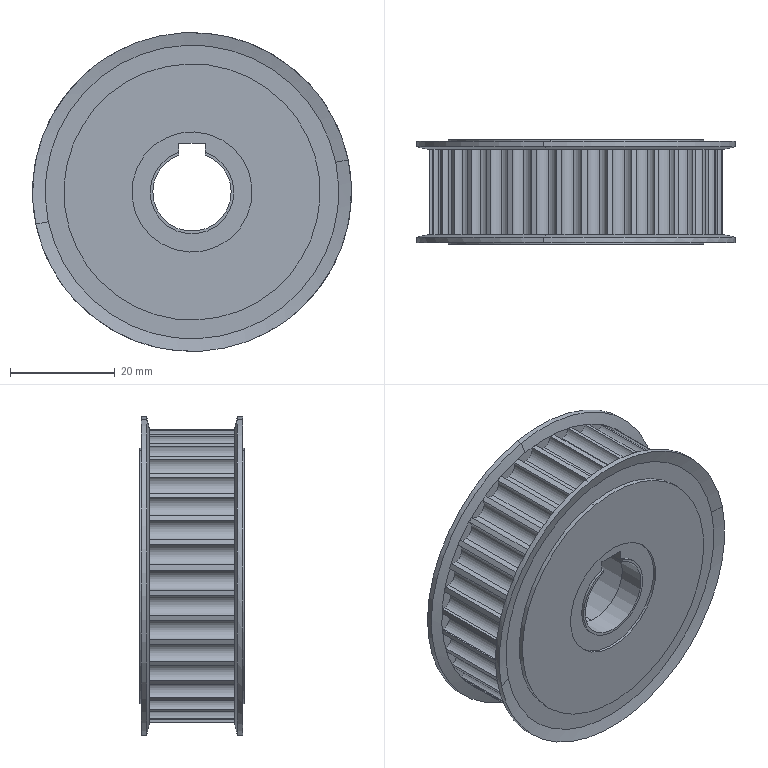Component | SolidWorks | ArcToothIdlerBearingTypeAtBothEnds[ST5GTD-36-15-Q]_ST5GTD-36-15-Q-1 | 1 solid | 133 faces | volume 40364 mm3 | cylinder 107 | plane 18 | cone 8 | commonest cylinder face diameters 3.86 x53 56.16 x36 49 x4 23 x4 61 x4 21.5 x2 16 x2 15 x2